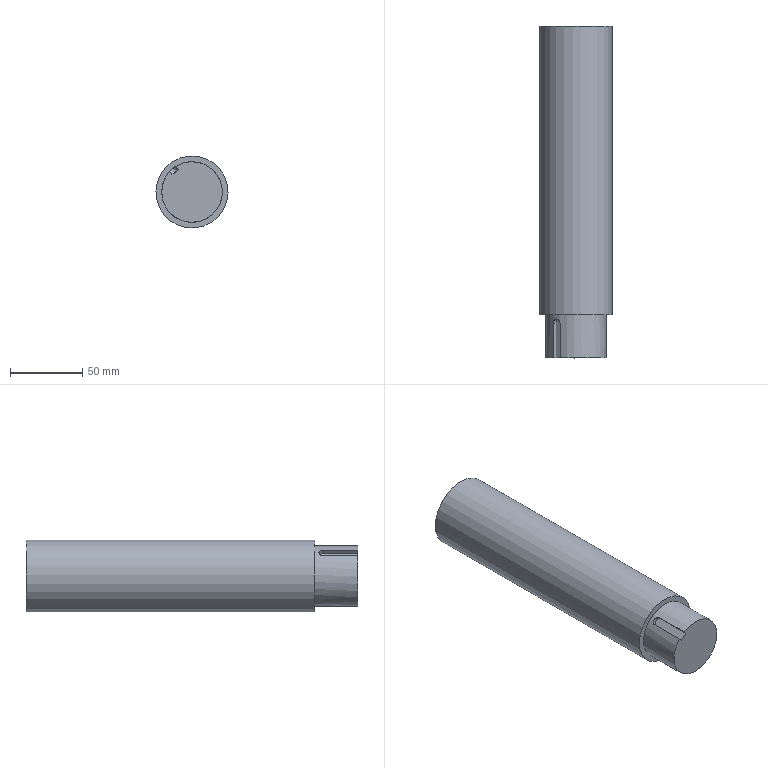Component | NX | MODEL2 | 2 solids | 10 faces | box 50 x 230 x 50 mm | volume 433799 mm3 | plane 7 | cylinder 3 | commonest cylinder face diameters 42 x1 6 x1 50 x1
STEP:
#1=CARTESIAN_POINT('',(0.,0.,0.));
#2=DIRECTION('',(0.,0.,1.));
#3=DIRECTION('',(1.,0.,0.));
#4=AXIS2_PLACEMENT_3D('',#1,#2,#3);
#5=CARTESIAN_POINT('',(848.938,50.431,-84.914));
#6=VERTEX_POINT('',#5);
#7=CARTESIAN_POINT('',(876.087,50.431,-89.266));
#8=VERTEX_POINT('',#7);
#9=CARTESIAN_POINT('',(860.,50.431,-102.764));
#10=DIRECTION('',(0.,1.,0.));
#11=DIRECTION('',(0.766,0.,0.6428));
#12=AXIS2_PLACEMENT_3D('',#9,#10,#11);
#13=CIRCLE('',#12,21.);
#14=CARTESIAN_POINT('',(860.,20.431,-102.764));
#15=DIRECTION('',(0.,1.,0.));
#16=DIRECTION('',(-0.6428,0.,0.766));
#17=AXIS2_PLACEMENT_3D('',#14,#15,#16);
#18=CYLINDRICAL_SURFACE('',#17,21.);
#19=CARTESIAN_POINT('',(-4.712,30.));
#20=DIRECTION('',(1.,0.));
#21=VECTOR('',#20,1.);
#22=LINE('',#19,#21);
#23=(GEOMETRIC_REPRESENTATION_CONTEXT(2)PARAMETRIC_REPRESENTATION_CONTEXT()REPRESENTATION_CONTEXT('',''));
#24=DEFINITIONAL_REPRESENTATION('',(#22),#23);
#25=PCURVE('',#18,#24);
#26=CARTESIAN_POINT('',(860.,50.431,-102.764));
#27=DIRECTION('',(0.,1.,0.));
#28=DIRECTION('',(-0.6428,0.,0.766));
#29=AXIS2_PLACEMENT_3D('',#26,#27,#28);
#30=PLANE('',#29);
#31=CARTESIAN_POINT('',(0.,0.));
#32=DIRECTION('',(0.,1.));
#33=AXIS2_PLACEMENT_2D('',#31,#32);
#34=CIRCLE('',#33,21.);
#35=(GEOMETRIC_REPRESENTATION_CONTEXT(2)PARAMETRIC_REPRESENTATION_CONTEXT()REPRESENTATION_CONTEXT('',''));
#36=DEFINITIONAL_REPRESENTATION('',(#34),#35);
#37=PCURVE('',#30,#36);
#38=SURFACE_CURVE('',#13,(#25,#37),.PCURVE_S1.);
#39=EDGE_CURVE('',#6,#8,#38,.T.);
#40=ORIENTED_EDGE('',*,*,#39,.F.);
#41=CARTESIAN_POINT('',(848.938,44.431,-84.914));
#42=VERTEX_POINT('',#41);
#43=CARTESIAN_POINT('',(848.938,44.431,-84.914));
#44=CARTESIAN_POINT('',(848.938,50.431,-84.914));
#45=B_SPLINE_CURVE_WITH_KNOTS('',1,(#43,#44),.UNSPECIFIED.,.F.,.F.,(2,2),(24.,30.),.PIECEWISE_BEZIER_KNOTS.);
#46=CARTESIAN_POINT('',(0.1433,0.));
#47=DIRECTION('',(0.,1.));
#48=VECTOR('',#47,1.);
#49=LINE('',#46,#48);
#50=(GEOMETRIC_REPRESENTATION_CONTEXT(2)PARAMETRIC_REPRESENTATION_CONTEXT()REPRESENTATION_CONTEXT('',''));
#51=DEFINITIONAL_REPRESENTATION('',(#49),#50);
#52=PCURVE('',#18,#51);
#53=CARTESIAN_POINT('',(6.427,0.));
#54=DIRECTION('',(0.,1.));
#55=VECTOR('',#54,1.);
#56=LINE('',#53,#55);
#57=(GEOMETRIC_REPRESENTATION_CONTEXT(2)PARAMETRIC_REPRESENTATION_CONTEXT()REPRESENTATION_CONTEXT('',''));
#58=DEFINITIONAL_REPRESENTATION('',(#56),#57);
#59=PCURVE('',#18,#58);
#60=SEAM_CURVE('',#45,(#52,#59),.PCURVE_S1.);
#61=EDGE_CURVE('',#42,#6,#60,.T.);
#62=ORIENTED_EDGE('',*,*,#61,.F.);
#63=CARTESIAN_POINT('',(848.938,20.431,-84.914));
#64=VERTEX_POINT('',#63);
#65=CARTESIAN_POINT('',(848.938,20.431,-84.914));
#66=DIRECTION('',(0.,-1.,0.));
#67=VECTOR('',#66,1.);
#68=LINE('',#65,#67);
#69=CARTESIAN_POINT('',(0.1433,0.));
#70=DIRECTION('',(0.,-1.));
#71=VECTOR('',#70,1.);
#72=LINE('',#69,#71);
#73=(GEOMETRIC_REPRESENTATION_CONTEXT(2)PARAMETRIC_REPRESENTATION_CONTEXT()REPRESENTATION_CONTEXT('',''));
#74=DEFINITIONAL_REPRESENTATION('',(#72),#73);
#75=PCURVE('',#18,#74);
#76=CARTESIAN_POINT('',(847.514,47.431,-83.217));
#77=DIRECTION('',(-0.766,0.,-0.6428));
#78=DIRECTION('',(-0.6428,0.,0.766));
#79=AXIS2_PLACEMENT_3D('',#76,#77,#78);
#80=PLANE('',#79);
#81=CARTESIAN_POINT('',(-2.215,-27.));
#82=DIRECTION('',(0.,-1.));
#83=VECTOR('',#82,1.);
#84=LINE('',#81,#83);
#85=(GEOMETRIC_REPRESENTATION_CONTEXT(2)PARAMETRIC_REPRESENTATION_CONTEXT()REPRESENTATION_CONTEXT('',''));
#86=DEFINITIONAL_REPRESENTATION('',(#84),#85);
#87=PCURVE('',#80,#86);
#88=SURFACE_CURVE('',#68,(#75,#87),.PCURVE_S1.);
#89=EDGE_CURVE('',#42,#64,#88,.T.);
#90=ORIENTED_EDGE('',*,*,#89,.T.);
#91=CARTESIAN_POINT('',(844.342,20.431,-88.771));
#92=VERTEX_POINT('',#91);
#93=CARTESIAN_POINT('',(860.,20.431,-102.764));
#94=DIRECTION('',(0.,1.,0.));
#95=DIRECTION('',(0.766,0.,0.6428));
#96=AXIS2_PLACEMENT_3D('',#93,#94,#95);
#97=CIRCLE('',#96,21.);
#98=CARTESIAN_POINT('',(-4.712,0.));
#99=DIRECTION('',(1.,0.));
#100=VECTOR('',#99,1.);
#101=LINE('',#98,#100);
#102=(GEOMETRIC_REPRESENTATION_CONTEXT(2)PARAMETRIC_REPRESENTATION_CONTEXT()REPRESENTATION_CONTEXT('',''));
#103=DEFINITIONAL_REPRESENTATION('',(#101),#102);
#104=PCURVE('',#18,#103);
#105=CARTESIAN_POINT('',(860.,20.431,-102.764));
#106=DIRECTION('',(0.,1.,0.));
#107=DIRECTION('',(-0.6428,0.,0.766));
#108=AXIS2_PLACEMENT_3D('',#105,#106,#107);
#109=PLANE('',#108);
#110=CARTESIAN_POINT('',(0.,0.));
#111=DIRECTION('',(0.,1.));
#112=AXIS2_PLACEMENT_2D('',#110,#111);
#113=CIRCLE('',#112,21.);
#114=(GEOMETRIC_REPRESENTATION_CONTEXT(2)PARAMETRIC_REPRESENTATION_CONTEXT()REPRESENTATION_CONTEXT('',''));
#115=DEFINITIONAL_REPRESENTATION('',(#113),#114);
#116=PCURVE('',#109,#115);
#117=SURFACE_CURVE('',#97,(#104,#116),.PCURVE_S1.);
#118=EDGE_CURVE('',#64,#92,#117,.T.);
#119=ORIENTED_EDGE('',*,*,#118,.T.);
#120=CARTESIAN_POINT('',(844.342,44.431,-88.771));
#121=VERTEX_POINT('',#120);
#122=CARTESIAN_POINT('',(844.342,20.431,-88.771));
#123=DIRECTION('',(0.,1.,0.));
#124=VECTOR('',#123,1.);
#125=LINE('',#122,#124);
#126=CARTESIAN_POINT('',(6.14,0.));
#127=DIRECTION('',(0.,1.));
#128=VECTOR('',#127,1.);
#129=LINE('',#126,#128);
#130=(GEOMETRIC_REPRESENTATION_CONTEXT(2)PARAMETRIC_REPRESENTATION_CONTEXT()REPRESENTATION_CONTEXT('',''));
#131=DEFINITIONAL_REPRESENTATION('',(#129),#130);
#132=PCURVE('',#18,#131);
#133=CARTESIAN_POINT('',(846.132,47.431,-90.904));
#134=DIRECTION('',(0.766,0.,0.6428));
#135=DIRECTION('',(0.6428,0.,-0.766));
#136=AXIS2_PLACEMENT_3D('',#133,#134,#135);
#137=PLANE('',#136);
#138=CARTESIAN_POINT('',(-2.785,-27.));
#139=DIRECTION('',(0.,1.));
#140=VECTOR('',#139,1.);
#141=LINE('',#138,#140);
#142=(GEOMETRIC_REPRESENTATION_CONTEXT(2)PARAMETRIC_REPRESENTATION_CONTEXT()REPRESENTATION_CONTEXT('',''));
#143=DEFINITIONAL_REPRESENTATION('',(#141),#142);
#144=PCURVE('',#137,#143);
#145=SURFACE_CURVE('',#125,(#132,#144),.PCURVE_S1.);
#146=EDGE_CURVE('',#92,#121,#145,.T.);
#147=ORIENTED_EDGE('',*,*,#146,.T.);
#148=CARTESIAN_POINT('',(844.342,44.431,-88.771));
#149=CARTESIAN_POINT('',(844.342,44.764,-88.771));
#150=CARTESIAN_POINT('',(844.38,45.103,-88.727));
#151=CARTESIAN_POINT('',(844.455,45.418,-88.645));
#152=CARTESIAN_POINT('',(844.529,45.733,-88.563));
#153=CARTESIAN_POINT('',(844.642,46.033,-88.441));
#154=CARTESIAN_POINT('',(844.785,46.294,-88.29));
#155=CARTESIAN_POINT('',(844.929,46.556,-88.138));
#156=CARTESIAN_POINT('',(845.109,46.787,-87.954));
#157=CARTESIAN_POINT('',(845.312,46.966,-87.755));
#158=CARTESIAN_POINT('',(845.516,47.146,-87.556));
#159=CARTESIAN_POINT('',(845.75,47.279,-87.336));
#160=CARTESIAN_POINT('',(845.995,47.355,-87.117));
#161=CARTESIAN_POINT('',(846.158,47.405,-86.97));
#162=CARTESIAN_POINT('',(846.329,47.431,-86.822));
#163=CARTESIAN_POINT('',(846.501,47.431,-86.677));
#164=CARTESIAN_POINT('',(846.757,47.431,-86.463));
#165=CARTESIAN_POINT('',(847.022,47.373,-86.252));
#166=CARTESIAN_POINT('',(847.273,47.264,-86.061));
#167=CARTESIAN_POINT('',(847.523,47.154,-85.869));
#168=CARTESIAN_POINT('',(847.767,46.989,-85.693));
#169=CARTESIAN_POINT('',(847.982,46.782,-85.543));
#170=CARTESIAN_POINT('',(848.198,46.574,-85.392));
#171=CARTESIAN_POINT('',(848.391,46.318,-85.264));
#172=CARTESIAN_POINT('',(848.542,46.034,-85.165));
#173=CARTESIAN_POINT('',(848.694,45.75,-85.066));
#174=CARTESIAN_POINT('',(848.808,45.43,-84.995));
#175=CARTESIAN_POINT('',(848.873,45.101,-84.955));
#176=CARTESIAN_POINT('',(848.916,44.882,-84.928));
#177=CARTESIAN_POINT('',(848.938,44.656,-84.914));
#178=CARTESIAN_POINT('',(848.938,44.431,-84.914));
#179=B_SPLINE_CURVE_WITH_KNOTS('',3,(#148,#149,#150,#151,#152,#153,#154,#155,#156,#157,#158,#159,#160,#161,#162,#163,#164,#165,#166,#167,#168,#169,#170,#171,#172,#173,#174,#175,#176,#177,#178),.UNSPECIFIED.,.F.,.F.,(4,3,3,3,3,3,3,3,3,3,4),(0.,0.1067,0.2134,0.3208,0.4286,0.5,0.6067,0.7134,0.8208,0.9286,1.),.UNSPECIFIED.);
#180=CARTESIAN_POINT('',(6.14,24.));
#181=CARTESIAN_POINT('',(6.14,24.071));
#182=CARTESIAN_POINT('',(6.14,24.214));
#183=CARTESIAN_POINT('',(6.141,24.427));
#184=CARTESIAN_POINT('',(6.143,24.639));
#185=CARTESIAN_POINT('',(6.146,24.847));
#186=CARTESIAN_POINT('',(6.149,25.049));
#187=CARTESIAN_POINT('',(6.153,25.247));
#188=CARTESIAN_POINT('',(6.157,25.439));
#189=CARTESIAN_POINT('',(6.163,25.623));
#190=CARTESIAN_POINT('',(6.168,25.799));
#191=CARTESIAN_POINT('',(6.175,25.965));
#192=CARTESIAN_POINT('',(6.182,26.121));
#193=CARTESIAN_POINT('',(6.189,26.268));
#194=CARTESIAN_POINT('',(6.197,26.402));
#195=CARTESIAN_POINT('',(6.206,26.524));
#196=CARTESIAN_POINT('',(6.214,26.633));
#197=CARTESIAN_POINT('',(6.224,26.729));
#198=CARTESIAN_POINT('',(6.233,26.812));
#199=CARTESIAN_POINT('',(6.243,26.88));
#200=CARTESIAN_POINT('',(6.253,26.933));
#201=CARTESIAN_POINT('',(6.263,26.972));
#202=CARTESIAN_POINT('',(6.273,26.995));
#203=CARTESIAN_POINT('',(6.283,27.003));
#204=CARTESIAN_POINT('',(6.293,26.995));
#205=CARTESIAN_POINT('',(6.304,26.972));
#206=CARTESIAN_POINT('',(6.314,26.934));
#207=CARTESIAN_POINT('',(6.324,26.881));
#208=CARTESIAN_POINT('',(6.333,26.813));
#209=CARTESIAN_POINT('',(6.343,26.731));
#210=CARTESIAN_POINT('',(6.352,26.635));
#211=CARTESIAN_POINT('',(6.361,26.526));
#212=CARTESIAN_POINT('',(6.369,26.404));
#213=CARTESIAN_POINT('',(6.377,26.27));
#214=CARTESIAN_POINT('',(6.384,26.124));
#215=CARTESIAN_POINT('',(6.391,25.967));
#216=CARTESIAN_POINT('',(6.398,25.801));
#217=CARTESIAN_POINT('',(6.404,25.626));
#218=CARTESIAN_POINT('',(6.409,25.442));
#219=CARTESIAN_POINT('',(6.414,25.251));
#220=CARTESIAN_POINT('',(6.417,25.052));
#221=CARTESIAN_POINT('',(6.421,24.849));
#222=CARTESIAN_POINT('',(6.423,24.642));
#223=CARTESIAN_POINT('',(6.425,24.43));
#224=CARTESIAN_POINT('',(6.426,24.215));
#225=CARTESIAN_POINT('',(6.427,24.072));
#226=CARTESIAN_POINT('',(6.427,24.));
#227=B_SPLINE_CURVE_WITH_KNOTS('',3,(#180,#181,#182,#183,#184,#185,#186,#187,#188,#189,#190,#191,#192,#193,#194,#195,#196,#197,#198,#199,#200,#201,#202,#203,#204,#205,#206,#207,#208,#209,#210,#211,#212,#213,#214,#215,#216,#217,#218,#219,#220,#221,#222,#223,#224,#225,#226),.UNSPECIFIED.,.F.,.F.,(4,1,1,1,1,1,1,1,1,1,1,1,1,1,1,1,1,1,1,1,1,1,1,1,1,1,1,1,1,1,1,1,1,1,1,1,1,1,1,1,1,1,1,1,4),(0.,0.02273,0.04545,0.06818,0.09091,0.1136,0.1364,0.1591,0.1818,0.2045,0.2273,0.25,0.2727,0.2955,0.3182,0.3409,0.3636,0.3864,0.4091,0.4318,0.4545,0.4773,0.5,0.5227,0.5455,0.5682,0.5909,0.6136,0.6364,0.6591,0.6818,0.7045,0.7273,0.75,0.7727,0.7955,0.8182,0.8409,0.8636,0.8864,0.9091,0.9318,0.9545,0.9773,1.),.QUASI_UNIFORM_KNOTS.);
#228=(GEOMETRIC_REPRESENTATION_CONTEXT(2)PARAMETRIC_REPRESENTATION_CONTEXT()REPRESENTATION_CONTEXT('',''));
#229=DEFINITIONAL_REPRESENTATION('',(#227),#228);
#230=PCURVE('',#18,#229);
#231=CARTESIAN_POINT('',(860.,44.431,-102.764));
#232=DIRECTION('',(0.6428,0.,-0.766));
#233=DIRECTION('',(-0.766,0.,-0.6428));
#234=AXIS2_PLACEMENT_3D('',#231,#232,#233);
#235=CYLINDRICAL_SURFACE('',#234,3.);
#236=CARTESIAN_POINT('',(0.,-20.785));
#237=CARTESIAN_POINT('',(0.0237,-20.785));
#238=CARTESIAN_POINT('',(0.07124,-20.785));
#239=CARTESIAN_POINT('',(0.1428,-20.789));
#240=CARTESIAN_POINT('',(0.2144,-20.794));
#241=CARTESIAN_POINT('',(0.2859,-20.802));
#242=CARTESIAN_POINT('',(0.3569,-20.811));
#243=CARTESIAN_POINT('',(0.4282,-20.822));
#244=CARTESIAN_POINT('',(0.4997,-20.834));
#245=CARTESIAN_POINT('',(0.5712,-20.848));
#246=CARTESIAN_POINT('',(0.6425,-20.862));
#247=CARTESIAN_POINT('',(0.7134,-20.877));
#248=CARTESIAN_POINT('',(0.7847,-20.892));
#249=CARTESIAN_POINT('',(0.8562,-20.908));
#250=CARTESIAN_POINT('',(0.9276,-20.923));
#251=CARTESIAN_POINT('',(0.9987,-20.937));
#252=CARTESIAN_POINT('',(1.07,-20.951));
#253=CARTESIAN_POINT('',(1.141,-20.963));
#254=CARTESIAN_POINT('',(1.213,-20.974));
#255=CARTESIAN_POINT('',(1.284,-20.983));
#256=CARTESIAN_POINT('',(1.355,-20.991));
#257=CARTESIAN_POINT('',(1.427,-20.996));
#258=CARTESIAN_POINT('',(1.499,-20.999));
#259=CARTESIAN_POINT('',(1.571,-21.));
#260=CARTESIAN_POINT('',(1.642,-20.999));
#261=CARTESIAN_POINT('',(1.714,-20.996));
#262=CARTESIAN_POINT('',(1.785,-20.991));
#263=CARTESIAN_POINT('',(1.857,-20.983));
#264=CARTESIAN_POINT('',(1.928,-20.974));
#265=CARTESIAN_POINT('',(1.999,-20.963));
#266=CARTESIAN_POINT('',(2.071,-20.951));
#267=CARTESIAN_POINT('',(2.142,-20.937));
#268=CARTESIAN_POINT('',(2.213,-20.923));
#269=CARTESIAN_POINT('',(2.284,-20.908));
#270=CARTESIAN_POINT('',(2.356,-20.893));
#271=CARTESIAN_POINT('',(2.427,-20.877));
#272=CARTESIAN_POINT('',(2.498,-20.862));
#273=CARTESIAN_POINT('',(2.57,-20.848));
#274=CARTESIAN_POINT('',(2.641,-20.834));
#275=CARTESIAN_POINT('',(2.712,-20.822));
#276=CARTESIAN_POINT('',(2.783,-20.811));
#277=CARTESIAN_POINT('',(2.855,-20.802));
#278=CARTESIAN_POINT('',(2.926,-20.794));
#279=CARTESIAN_POINT('',(2.998,-20.789));
#280=CARTESIAN_POINT('',(3.07,-20.785));
#281=CARTESIAN_POINT('',(3.118,-20.785));
#282=CARTESIAN_POINT('',(3.142,-20.785));
#283=B_SPLINE_CURVE_WITH_KNOTS('',3,(#236,#237,#238,#239,#240,#241,#242,#243,#244,#245,#246,#247,#248,#249,#250,#251,#252,#253,#254,#255,#256,#257,#258,#259,#260,#261,#262,#263,#264,#265,#266,#267,#268,#269,#270,#271,#272,#273,#274,#275,#276,#277,#278,#279,#280,#281,#282),.UNSPECIFIED.,.F.,.F.,(4,1,1,1,1,1,1,1,1,1,1,1,1,1,1,1,1,1,1,1,1,1,1,1,1,1,1,1,1,1,1,1,1,1,1,1,1,1,1,1,1,1,1,1,4),(0.,0.02273,0.04545,0.06818,0.09091,0.1136,0.1364,0.1591,0.1818,0.2045,0.2273,0.25,0.2727,0.2955,0.3182,0.3409,0.3636,0.3864,0.4091,0.4318,0.4545,0.4773,0.5,0.5227,0.5455,0.5682,0.5909,0.6136,0.6364,0.6591,0.6818,0.7045,0.7273,0.75,0.7727,0.7955,0.8182,0.8409,0.8636,0.8864,0.9091,0.9318,0.9545,0.9773,1.),.QUASI_UNIFORM_KNOTS.);
#284=(GEOMETRIC_REPRESENTATION_CONTEXT(2)PARAMETRIC_REPRESENTATION_CONTEXT()REPRESENTATION_CONTEXT('',''));
#285=DEFINITIONAL_REPRESENTATION('',(#283),#284);
#286=PCURVE('',#235,#285);
#287=SURFACE_CURVE('',#179,(#230,#286),.PCURVE_S1.);
#288=EDGE_CURVE('',#121,#42,#287,.T.);
#289=ORIENTED_EDGE('',*,*,#288,.T.);
#290=ORIENTED_EDGE('',*,*,#61,.T.);
#291=CARTESIAN_POINT('',(860.,50.431,-102.764));
#292=DIRECTION('',(0.,1.,0.));
#293=DIRECTION('',(0.766,0.,0.6428));
#294=AXIS2_PLACEMENT_3D('',#291,#292,#293);
#295=CIRCLE('',#294,21.);
#296=CARTESIAN_POINT('',(1.571,30.));
#297=DIRECTION('',(1.,0.));
#298=VECTOR('',#297,1.);
#299=LINE('',#296,#298);
#300=(GEOMETRIC_REPRESENTATION_CONTEXT(2)PARAMETRIC_REPRESENTATION_CONTEXT()REPRESENTATION_CONTEXT('',''));
#301=DEFINITIONAL_REPRESENTATION('',(#299),#300);
#302=PCURVE('',#18,#301);
#303=CARTESIAN_POINT('',(0.,0.));
#304=DIRECTION('',(0.,1.));
#305=AXIS2_PLACEMENT_2D('',#303,#304);
#306=CIRCLE('',#305,21.);
#307=(GEOMETRIC_REPRESENTATION_CONTEXT(2)PARAMETRIC_REPRESENTATION_CONTEXT()REPRESENTATION_CONTEXT('',''));
#308=DEFINITIONAL_REPRESENTATION('',(#306),#307);
#309=PCURVE('',#30,#308);
#310=SURFACE_CURVE('',#295,(#302,#309),.PCURVE_S1.);
#311=EDGE_CURVE('',#8,#6,#310,.T.);
#312=ORIENTED_EDGE('',*,*,#311,.F.);
#313=EDGE_LOOP('',(#40,#62,#90,#119,#147,#289,#290,#312));
#314=FACE_BOUND('',#313,.T.);
#315=ADVANCED_FACE('',(#314),#18,.T.);
#316=ORIENTED_EDGE('',*,*,#118,.F.);
#317=CARTESIAN_POINT('',(850.728,20.431,-87.047));
#318=VERTEX_POINT('',#317);
#319=CARTESIAN_POINT('',(847.514,20.431,-83.217));
#320=DIRECTION('',(0.6428,0.,-0.766));
#321=VECTOR('',#320,1.);
#322=LINE('',#319,#321);
#323=CARTESIAN_POINT('',(23.,3.));
#324=DIRECTION('',(-1.,0.));
#325=VECTOR('',#324,1.);
#326=LINE('',#323,#325);
#327=(GEOMETRIC_REPRESENTATION_CONTEXT(2)PARAMETRIC_REPRESENTATION_CONTEXT()REPRESENTATION_CONTEXT('',''));
#328=DEFINITIONAL_REPRESENTATION('',(#326),#327);
#329=PCURVE('',#109,#328);
#330=CARTESIAN_POINT('',(0.,-27.));
#331=DIRECTION('',(-1.,0.));
#332=VECTOR('',#331,1.);
#333=LINE('',#330,#332);
#334=(GEOMETRIC_REPRESENTATION_CONTEXT(2)PARAMETRIC_REPRESENTATION_CONTEXT()REPRESENTATION_CONTEXT('',''));
#335=DEFINITIONAL_REPRESENTATION('',(#333),#334);
#336=PCURVE('',#80,#335);
#337=SURFACE_CURVE('',#322,(#329,#336),.PCURVE_S1.);
#338=EDGE_CURVE('',#64,#318,#337,.T.);
#339=ORIENTED_EDGE('',*,*,#338,.T.);
#340=CARTESIAN_POINT('',(846.132,20.431,-90.904));
#341=VERTEX_POINT('',#340);
#342=CARTESIAN_POINT('',(850.728,20.431,-87.047));
#343=DIRECTION('',(-0.766,0.,-0.6428));
#344=VECTOR('',#343,1.);
#345=LINE('',#342,#344);
#346=CARTESIAN_POINT('',(18.,3.));
#347=DIRECTION('',(0.,-1.));
#348=VECTOR('',#347,1.);
#349=LINE('',#346,#348);
#350=(GEOMETRIC_REPRESENTATION_CONTEXT(2)PARAMETRIC_REPRESENTATION_CONTEXT()REPRESENTATION_CONTEXT('',''));
#351=DEFINITIONAL_REPRESENTATION('',(#349),#350);
#352=PCURVE('',#109,#351);
#353=CARTESIAN_POINT('',(850.728,47.431,-87.047));
#354=DIRECTION('',(-0.6428,0.,0.766));
#355=DIRECTION('',(0.766,0.,0.6428));
#356=AXIS2_PLACEMENT_3D('',#353,#354,#355);
#357=PLANE('',#356);
#358=CARTESIAN_POINT('',(0.,-27.));
#359=DIRECTION('',(-1.,0.));
#360=VECTOR('',#359,1.);
#361=LINE('',#358,#360);
#362=(GEOMETRIC_REPRESENTATION_CONTEXT(2)PARAMETRIC_REPRESENTATION_CONTEXT()REPRESENTATION_CONTEXT('',''));
#363=DEFINITIONAL_REPRESENTATION('',(#361),#362);
#364=PCURVE('',#357,#363);
#365=SURFACE_CURVE('',#345,(#352,#364),.PCURVE_S1.);
#366=EDGE_CURVE('',#318,#341,#365,.T.);
#367=ORIENTED_EDGE('',*,*,#366,.T.);
#368=CARTESIAN_POINT('',(846.132,20.431,-90.904));
#369=DIRECTION('',(-0.6428,0.,0.766));
#370=VECTOR('',#369,1.);
#371=LINE('',#368,#370);
#372=CARTESIAN_POINT('',(18.,-3.));
#373=DIRECTION('',(1.,0.));
#374=VECTOR('',#373,1.);
#375=LINE('',#372,#374);
#376=(GEOMETRIC_REPRESENTATION_CONTEXT(2)PARAMETRIC_REPRESENTATION_CONTEXT()REPRESENTATION_CONTEXT('',''));
#377=DEFINITIONAL_REPRESENTATION('',(#375),#376);
#378=PCURVE('',#109,#377);
#379=CARTESIAN_POINT('',(0.,-27.));
#380=DIRECTION('',(-1.,0.));
#381=VECTOR('',#380,1.);
#382=LINE('',#379,#381);
#383=(GEOMETRIC_REPRESENTATION_CONTEXT(2)PARAMETRIC_REPRESENTATION_CONTEXT()REPRESENTATION_CONTEXT('',''));
#384=DEFINITIONAL_REPRESENTATION('',(#382),#383);
#385=PCURVE('',#137,#384);
#386=SURFACE_CURVE('',#371,(#378,#385),.PCURVE_S1.);
#387=EDGE_CURVE('',#341,#92,#386,.T.);
#388=ORIENTED_EDGE('',*,*,#387,.T.);
#389=EDGE_LOOP('',(#316,#339,#367,#388));
#390=FACE_BOUND('',#389,.T.);
#391=ADVANCED_FACE('',(#390),#109,.F.);
#392=ORIENTED_EDGE('',*,*,#311,.T.);
#393=ORIENTED_EDGE('',*,*,#39,.T.);
#394=EDGE_LOOP('',(#392,#393));
#395=FACE_BOUND('',#394,.T.);
#396=ADVANCED_FACE('',(#395),#30,.T.);
#397=ORIENTED_EDGE('',*,*,#89,.F.);
#398=CARTESIAN_POINT('',(850.728,44.431,-87.047));
#399=VERTEX_POINT('',#398);
#400=CARTESIAN_POINT('',(847.514,44.431,-83.217));
#401=DIRECTION('',(0.6428,0.,-0.766));
#402=VECTOR('',#401,1.);
#403=LINE('',#400,#402);
#404=CARTESIAN_POINT('',(0.,-3.));
#405=DIRECTION('',(-1.,0.));
#406=VECTOR('',#405,1.);
#407=LINE('',#404,#406);
#408=(GEOMETRIC_REPRESENTATION_CONTEXT(2)PARAMETRIC_REPRESENTATION_CONTEXT()REPRESENTATION_CONTEXT('',''));
#409=DEFINITIONAL_REPRESENTATION('',(#407),#408);
#410=PCURVE('',#80,#409);
#411=CARTESIAN_POINT('',(3.142,-23.));
#412=DIRECTION('',(0.,1.));
#413=VECTOR('',#412,1.);
#414=LINE('',#411,#413);
#415=(GEOMETRIC_REPRESENTATION_CONTEXT(2)PARAMETRIC_REPRESENTATION_CONTEXT()REPRESENTATION_CONTEXT('',''));
#416=DEFINITIONAL_REPRESENTATION('',(#414),#415);
#417=PCURVE('',#235,#416);
#418=SURFACE_CURVE('',#403,(#410,#417),.PCURVE_S1.);
#419=EDGE_CURVE('',#42,#399,#418,.T.);
#420=ORIENTED_EDGE('',*,*,#419,.T.);
#421=CARTESIAN_POINT('',(850.728,47.431,-87.047));
#422=DIRECTION('',(0.,1.,0.));
#423=VECTOR('',#422,1.);
#424=LINE('',#421,#423);
#425=CARTESIAN_POINT('',(-5.,0.));
#426=DIRECTION('',(0.,1.));
#427=VECTOR('',#426,1.);
#428=LINE('',#425,#427);
#429=(GEOMETRIC_REPRESENTATION_CONTEXT(2)PARAMETRIC_REPRESENTATION_CONTEXT()REPRESENTATION_CONTEXT('',''));
#430=DEFINITIONAL_REPRESENTATION('',(#428),#429);
#431=PCURVE('',#80,#430);
#432=CARTESIAN_POINT('',(0.,0.));
#433=DIRECTION('',(0.,1.));
#434=VECTOR('',#433,1.);
#435=LINE('',#432,#434);
#436=(GEOMETRIC_REPRESENTATION_CONTEXT(2)PARAMETRIC_REPRESENTATION_CONTEXT()REPRESENTATION_CONTEXT('',''));
#437=DEFINITIONAL_REPRESENTATION('',(#435),#436);
#438=PCURVE('',#357,#437);
#439=SURFACE_CURVE('',#424,(#431,#438),.PCURVE_S1.);
#440=EDGE_CURVE('',#318,#399,#439,.T.);
#441=ORIENTED_EDGE('',*,*,#440,.F.);
#442=ORIENTED_EDGE('',*,*,#338,.F.);
#443=EDGE_LOOP('',(#397,#420,#441,#442));
#444=FACE_BOUND('',#443,.T.);
#445=ADVANCED_FACE('',(#444),#80,.T.);
#446=ORIENTED_EDGE('',*,*,#440,.T.);
#447=CARTESIAN_POINT('',(846.132,44.431,-90.904));
#448=VERTEX_POINT('',#447);
#449=CARTESIAN_POINT('',(848.43,44.431,-88.975));
#450=DIRECTION('',(-0.6428,0.,0.766));
#451=DIRECTION('',(0.766,0.,0.6428));
#452=AXIS2_PLACEMENT_3D('',#449,#450,#451);
#453=CIRCLE('',#452,3.);
#454=CARTESIAN_POINT('',(-3.,-3.));
#455=DIRECTION('',(1.,0.));
#456=AXIS2_PLACEMENT_2D('',#454,#455);
#457=CIRCLE('',#456,3.);
#458=(GEOMETRIC_REPRESENTATION_CONTEXT(2)PARAMETRIC_REPRESENTATION_CONTEXT()REPRESENTATION_CONTEXT('',''));
#459=DEFINITIONAL_REPRESENTATION('',(#457),#458);
#460=PCURVE('',#357,#459);
#461=CARTESIAN_POINT('',(3.142,-18.));
#462=DIRECTION('',(-1.,-0.));
#463=VECTOR('',#462,1.);
#464=LINE('',#461,#463);
#465=(GEOMETRIC_REPRESENTATION_CONTEXT(2)PARAMETRIC_REPRESENTATION_CONTEXT()REPRESENTATION_CONTEXT('',''));
#466=DEFINITIONAL_REPRESENTATION('',(#464),#465);
#467=PCURVE('',#235,#466);
#468=SURFACE_CURVE('',#453,(#460,#467),.PCURVE_S1.);
#469=EDGE_CURVE('',#399,#448,#468,.T.);
#470=ORIENTED_EDGE('',*,*,#469,.T.);
#471=CARTESIAN_POINT('',(846.132,47.431,-90.904));
#472=DIRECTION('',(0.,1.,0.));
#473=VECTOR('',#472,1.);
#474=LINE('',#471,#473);
#475=CARTESIAN_POINT('',(-6.,0.));
#476=DIRECTION('',(0.,1.));
#477=VECTOR('',#476,1.);
#478=LINE('',#475,#477);
#479=(GEOMETRIC_REPRESENTATION_CONTEXT(2)PARAMETRIC_REPRESENTATION_CONTEXT()REPRESENTATION_CONTEXT('',''));
#480=DEFINITIONAL_REPRESENTATION('',(#478),#479);
#481=PCURVE('',#357,#480);
#482=CARTESIAN_POINT('',(0.,0.));
#483=DIRECTION('',(0.,1.));
#484=VECTOR('',#483,1.);
#485=LINE('',#482,#484);
#486=(GEOMETRIC_REPRESENTATION_CONTEXT(2)PARAMETRIC_REPRESENTATION_CONTEXT()REPRESENTATION_CONTEXT('',''));
#487=DEFINITIONAL_REPRESENTATION('',(#485),#486);
#488=PCURVE('',#137,#487);
#489=SURFACE_CURVE('',#474,(#481,#488),.PCURVE_S1.);
#490=EDGE_CURVE('',#341,#448,#489,.T.);
#491=ORIENTED_EDGE('',*,*,#490,.F.);
#492=ORIENTED_EDGE('',*,*,#366,.F.);
#493=EDGE_LOOP('',(#446,#470,#491,#492));
#494=FACE_BOUND('',#493,.T.);
#495=ADVANCED_FACE('',(#494),#357,.T.);
#496=ORIENTED_EDGE('',*,*,#490,.T.);
#497=CARTESIAN_POINT('',(846.132,44.431,-90.904));
#498=DIRECTION('',(-0.6428,0.,0.766));
#499=VECTOR('',#498,1.);
#500=LINE('',#497,#499);
#501=CARTESIAN_POINT('',(0.,-3.));
#502=DIRECTION('',(-1.,0.));
#503=VECTOR('',#502,1.);
#504=LINE('',#501,#503);
#505=(GEOMETRIC_REPRESENTATION_CONTEXT(2)PARAMETRIC_REPRESENTATION_CONTEXT()REPRESENTATION_CONTEXT('',''));
#506=DEFINITIONAL_REPRESENTATION('',(#504),#505);
#507=PCURVE('',#137,#506);
#508=CARTESIAN_POINT('',(0.,-18.));
#509=DIRECTION('',(0.,-1.));
#510=VECTOR('',#509,1.);
#511=LINE('',#508,#510);
#512=(GEOMETRIC_REPRESENTATION_CONTEXT(2)PARAMETRIC_REPRESENTATION_CONTEXT()REPRESENTATION_CONTEXT('',''));
#513=DEFINITIONAL_REPRESENTATION('',(#511),#512);
#514=PCURVE('',#235,#513);
#515=SURFACE_CURVE('',#500,(#507,#514),.PCURVE_S1.);
#516=EDGE_CURVE('',#448,#121,#515,.T.);
#517=ORIENTED_EDGE('',*,*,#516,.T.);
#518=ORIENTED_EDGE('',*,*,#146,.F.);
#519=ORIENTED_EDGE('',*,*,#387,.F.);
#520=EDGE_LOOP('',(#496,#517,#518,#519));
#521=FACE_BOUND('',#520,.T.);
#522=ADVANCED_FACE('',(#521),#137,.T.);
#523=ORIENTED_EDGE('',*,*,#288,.T.);
#524=ORIENTED_EDGE('',*,*,#419,.T.);
#525=ORIENTED_EDGE('',*,*,#469,.T.);
#526=ORIENTED_EDGE('',*,*,#516,.T.);
#527=EDGE_LOOP('',(#523,#524,#525,#526));
#528=FACE_BOUND('',#527,.F.);
#529=ADVANCED_FACE('',(#528),#235,.F.);
#530=CLOSED_SHELL('',(#315,#391,#396,#445,#495,#522,#529));
#531=MANIFOLD_SOLID_BREP('',#530);
#532=(LENGTH_UNIT()NAMED_UNIT(*)SI_UNIT(.MILLI.,.METRE.));
#533=UNCERTAINTY_MEASURE_WITH_UNIT(LENGTH_MEASURE(0.00005),#532,'','');
#534=(NAMED_UNIT(*)PLANE_ANGLE_UNIT()SI_UNIT($,.RADIAN.));
#535=(NAMED_UNIT(*)SI_UNIT($,.STERADIAN.)SOLID_ANGLE_UNIT());
#536=(GEOMETRIC_REPRESENTATION_CONTEXT(3)GLOBAL_UNCERTAINTY_ASSIGNED_CONTEXT((#533))GLOBAL_UNIT_ASSIGNED_CONTEXT((#532,#534,#535))REPRESENTATION_CONTEXT('',''));
#537=ADVANCED_BREP_SHAPE_REPRESENTATION('',(#4,#531),#536);
#538=CARTESIAN_POINT('',(0.,0.,0.));
#539=DIRECTION('',(0.,0.,1.));
#540=DIRECTION('',(1.,0.,0.));
#541=AXIS2_PLACEMENT_3D('',#538,#539,#540);
#542=CARTESIAN_POINT('',(0.,0.,0.));
#543=DIRECTION('',(0.,0.,1.));
#544=DIRECTION('',(1.,0.,0.));
#545=AXIS2_PLACEMENT_3D('',#542,#543,#544);
#546=(LENGTH_UNIT()NAMED_UNIT(*)SI_UNIT(.MILLI.,.METRE.));
#547=UNCERTAINTY_MEASURE_WITH_UNIT(LENGTH_MEASURE(0.00005),#546,'','');
#548=(NAMED_UNIT(*)PLANE_ANGLE_UNIT()SI_UNIT($,.RADIAN.));
#549=(NAMED_UNIT(*)SI_UNIT($,.STERADIAN.)SOLID_ANGLE_UNIT());
#550=(GEOMETRIC_REPRESENTATION_CONTEXT(3)GLOBAL_UNCERTAINTY_ASSIGNED_CONTEXT((#547))GLOBAL_UNIT_ASSIGNED_CONTEXT((#546,#548,#549))REPRESENTATION_CONTEXT('',''));
#551=SHAPE_REPRESENTATION('',(#4,#541,#545),#550);
#552=ITEM_DEFINED_TRANSFORMATION('','',#4,#541);
#553=(REPRESENTATION_RELATIONSHIP('','',#537,#551)REPRESENTATION_RELATIONSHIP_WITH_TRANSFORMATION(#552)SHAPE_REPRESENTATION_RELATIONSHIP());
#554=CARTESIAN_POINT('',(879.151,250.431,-86.695));
#555=VERTEX_POINT('',#554);
#556=CARTESIAN_POINT('',(860.,250.431,-102.764));
#557=DIRECTION('',(0.,-1.,0.));
#558=DIRECTION('',(0.766,0.,0.6428));
#559=AXIS2_PLACEMENT_3D('',#556,#557,#558);
#560=CIRCLE('',#559,25.);
#561=CARTESIAN_POINT('',(860.,250.431,-102.764));
#562=DIRECTION('',(0.,-1.,0.));
#563=DIRECTION('',(0.6428,0.,-0.766));
#564=AXIS2_PLACEMENT_3D('',#561,#562,#563);
#565=CYLINDRICAL_SURFACE('',#564,25.);
#566=CARTESIAN_POINT('',(1.571,0.));
#567=DIRECTION('',(1.,0.));
#568=VECTOR('',#567,1.);
#569=LINE('',#566,#568);
#570=(GEOMETRIC_REPRESENTATION_CONTEXT(2)PARAMETRIC_REPRESENTATION_CONTEXT()REPRESENTATION_CONTEXT('',''));
#571=DEFINITIONAL_REPRESENTATION('',(#569),#570);
#572=PCURVE('',#565,#571);
#573=CARTESIAN_POINT('',(860.,250.431,-102.764));
#574=DIRECTION('',(0.,-1.,0.));
#575=DIRECTION('',(0.6428,0.,-0.766));
#576=AXIS2_PLACEMENT_3D('',#573,#574,#575);
#577=PLANE('',#576);
#578=CARTESIAN_POINT('',(0.,0.));
#579=DIRECTION('',(0.,1.));
#580=AXIS2_PLACEMENT_2D('',#578,#579);
#581=CIRCLE('',#580,25.);
#582=(GEOMETRIC_REPRESENTATION_CONTEXT(2)PARAMETRIC_REPRESENTATION_CONTEXT()REPRESENTATION_CONTEXT('',''));
#583=DEFINITIONAL_REPRESENTATION('',(#581),#582);
#584=PCURVE('',#577,#583);
#585=SURFACE_CURVE('',#560,(#572,#584),.PCURVE_S1.);
#586=EDGE_CURVE('',#555,#555,#585,.T.);
#587=ORIENTED_EDGE('',*,*,#586,.T.);
#588=CARTESIAN_POINT('',(879.151,50.431,-86.695));
#589=VERTEX_POINT('',#588);
#590=CARTESIAN_POINT('',(879.151,250.431,-86.695));
#591=CARTESIAN_POINT('',(879.151,50.431,-86.695));
#592=B_SPLINE_CURVE_WITH_KNOTS('',1,(#590,#591),.UNSPECIFIED.,.F.,.F.,(2,2),(0.,200.),.PIECEWISE_BEZIER_KNOTS.);
#593=CARTESIAN_POINT('',(7.854,0.));
#594=DIRECTION('',(0.,1.));
#595=VECTOR('',#594,1.);
#596=LINE('',#593,#595);
#597=(GEOMETRIC_REPRESENTATION_CONTEXT(2)PARAMETRIC_REPRESENTATION_CONTEXT()REPRESENTATION_CONTEXT('',''));
#598=DEFINITIONAL_REPRESENTATION('',(#596),#597);
#599=PCURVE('',#565,#598);
#600=CARTESIAN_POINT('',(1.571,0.));
#601=DIRECTION('',(0.,1.));
#602=VECTOR('',#601,1.);
#603=LINE('',#600,#602);
#604=(GEOMETRIC_REPRESENTATION_CONTEXT(2)PARAMETRIC_REPRESENTATION_CONTEXT()REPRESENTATION_CONTEXT('',''));
#605=DEFINITIONAL_REPRESENTATION('',(#603),#604);
#606=PCURVE('',#565,#605);
#607=SEAM_CURVE('',#592,(#599,#606),.PCURVE_S1.);
#608=EDGE_CURVE('',#555,#589,#607,.T.);
#609=ORIENTED_EDGE('',*,*,#608,.T.);
#610=CARTESIAN_POINT('',(860.,50.431,-102.764));
#611=DIRECTION('',(0.,-1.,0.));
#612=DIRECTION('',(0.766,0.,0.6428));
#613=AXIS2_PLACEMENT_3D('',#610,#611,#612);
#614=CIRCLE('',#613,25.);
#615=CARTESIAN_POINT('',(1.571,200.));
#616=DIRECTION('',(1.,0.));
#617=VECTOR('',#616,1.);
#618=LINE('',#615,#617);
#619=(GEOMETRIC_REPRESENTATION_CONTEXT(2)PARAMETRIC_REPRESENTATION_CONTEXT()REPRESENTATION_CONTEXT('',''));
#620=DEFINITIONAL_REPRESENTATION('',(#618),#619);
#621=PCURVE('',#565,#620);
#622=CARTESIAN_POINT('',(860.,50.431,-102.764));
#623=DIRECTION('',(0.,-1.,0.));
#624=DIRECTION('',(0.6428,0.,-0.766));
#625=AXIS2_PLACEMENT_3D('',#622,#623,#624);
#626=PLANE('',#625);
#627=CARTESIAN_POINT('',(0.,0.));
#628=DIRECTION('',(0.,1.));
#629=AXIS2_PLACEMENT_2D('',#627,#628);
#630=CIRCLE('',#629,25.);
#631=(GEOMETRIC_REPRESENTATION_CONTEXT(2)PARAMETRIC_REPRESENTATION_CONTEXT()REPRESENTATION_CONTEXT('',''));
#632=DEFINITIONAL_REPRESENTATION('',(#630),#631);
#633=PCURVE('',#626,#632);
#634=SURFACE_CURVE('',#614,(#621,#633),.PCURVE_S1.);
#635=EDGE_CURVE('',#589,#589,#634,.T.);
#636=ORIENTED_EDGE('',*,*,#635,.F.);
#637=ORIENTED_EDGE('',*,*,#608,.F.);
#638=EDGE_LOOP('',(#587,#609,#636,#637));
#639=FACE_BOUND('',#638,.T.);
#640=ADVANCED_FACE('',(#639),#565,.T.);
#641=ORIENTED_EDGE('',*,*,#586,.F.);
#642=EDGE_LOOP('',(#641));
#643=FACE_BOUND('',#642,.T.);
#644=ADVANCED_FACE('',(#643),#577,.F.);
#645=ORIENTED_EDGE('',*,*,#635,.T.);
#646=EDGE_LOOP('',(#645));
#647=FACE_BOUND('',#646,.T.);
#648=ADVANCED_FACE('',(#647),#626,.T.);
#649=CLOSED_SHELL('',(#640,#644,#648));
#650=MANIFOLD_SOLID_BREP('',#649);
#651=(LENGTH_UNIT()NAMED_UNIT(*)SI_UNIT(.MILLI.,.METRE.));
#652=UNCERTAINTY_MEASURE_WITH_UNIT(LENGTH_MEASURE(0.00001),#651,'','');
#653=(NAMED_UNIT(*)PLANE_ANGLE_UNIT()SI_UNIT($,.RADIAN.));
#654=(NAMED_UNIT(*)SI_UNIT($,.STERADIAN.)SOLID_ANGLE_UNIT());
#655=(GEOMETRIC_REPRESENTATION_CONTEXT(3)GLOBAL_UNCERTAINTY_ASSIGNED_CONTEXT((#652))GLOBAL_UNIT_ASSIGNED_CONTEXT((#651,#653,#654))REPRESENTATION_CONTEXT('',''));
#656=ADVANCED_BREP_SHAPE_REPRESENTATION('',(#4,#650),#655);
#657=ITEM_DEFINED_TRANSFORMATION('','',#4,#545);
#658=(REPRESENTATION_RELATIONSHIP('','',#656,#551)REPRESENTATION_RELATIONSHIP_WITH_TRANSFORMATION(#657)SHAPE_REPRESENTATION_RELATIONSHIP());